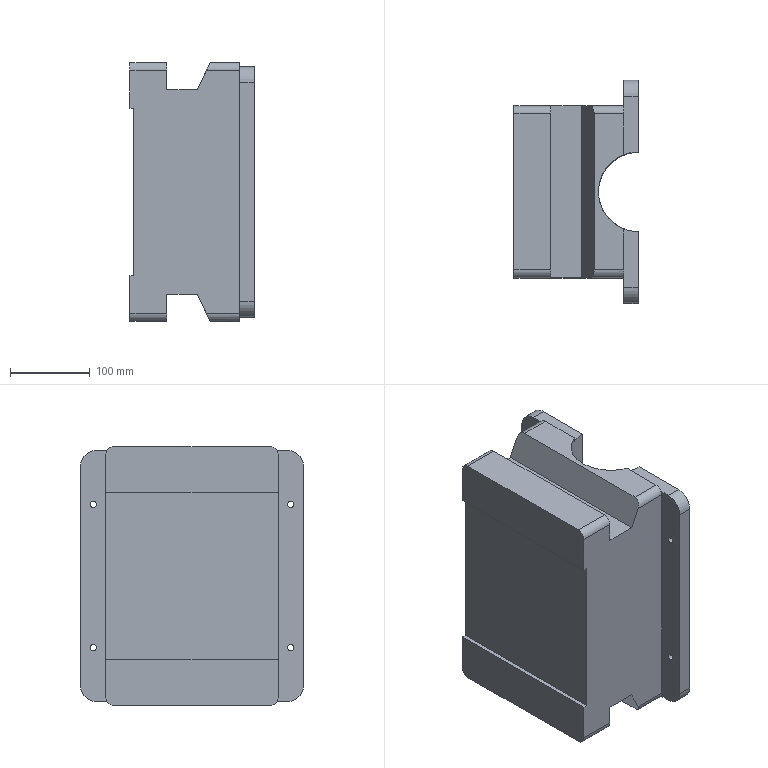Component | SolidWorks | Box-1 | 1 solid | 74 faces | box 156 x 280 x 325 mm | volume 4058266 mm3 | plane 40 | cylinder 34 | commonest cylinder face diameters 12 x8 8 x8 20 x8 40 x8 100 x2
build123d program:
from build123d import *

# Parameters (mm, degrees)
BOSS_EXTRUDE1_DEPTH = 18
BOSS_EXTRUDE2_DEPTH = 138
CUT_EXTRUDE1_DEPTH  = 141
CUT_EXTRUDE2_DEPTH  = 336.032
CUT_EXTRUDE3_DEPTH  = 336.032
CUT_EXTRUDE4_DEPTH  = 500
SKETCH7_R           = 4
SKETCH7_R_2         = 6
CUT_EXTRUDE5_DEPTH  = 20


with BuildPart() as part:
    # Sketch1 → Boss-Extrude1 (new body)
    with BuildSketch(Plane(origin=(0, 0, 0), x_dir=(0, 0, -1), z_dir=(1, 0, 0))):
        with BuildLine():
            Line((137.5, 140), (-137.5, 140))
            ThreePointArc((-137.5, 140), (-151.642, 134.142), (-157.5, 120))
            Line((-157.5, 120), (-157.5, -120))
            ThreePointArc((-157.5, -120), (-151.642, -134.142), (-137.5, -140))
            Line((-137.5, -140), (137.5, -140))
            ThreePointArc((137.5, -140), (151.642, -134.142), (157.5, -120))
            Line((157.5, -120), (157.5, 120))
            ThreePointArc((157.5, 120), (151.642, 134.142), (137.5, 140))
        make_face()
    extrude(amount=BOSS_EXTRUDE1_DEPTH)

    # Sketch2 → Boss-Extrude2 (add)
    with BuildSketch(Plane(origin=(18, 0, 0), x_dir=(0, 0, -1), z_dir=(1, 0, 0))):
        with BuildLine():
            Line((152.5, 108), (-152.5, 108))
            ThreePointArc((-152.5, 108), (-159.571, 105.071), (-162.5, 98))
            Line((-162.5, 98), (-162.5, -98))
            ThreePointArc((-162.5, -98), (-159.571, -105.071), (-152.5, -108))
            Line((-152.5, -108), (152.5, -108))
            ThreePointArc((152.5, -108), (159.571, -105.071), (162.5, -98))
            Line((162.5, -98), (162.5, 98))
            ThreePointArc((162.5, 98), (159.571, 105.071), (152.5, 108))
        make_face()
    extrude(amount=BOSS_EXTRUDE2_DEPTH)

    # Sketch3 → Cut-Extrude1 (cut)
    with BuildSketch(Plane.ZY):
        with BuildLine():
            Line((89.5, 96), (-89.5, 96))
            ThreePointArc((-89.5, 96), (-103.642, 90.142), (-109.5, 76))
            Line((-109.5, 76), (-109.5, -76))
            ThreePointArc((-109.5, -76), (-103.642, -90.142), (-89.5, -96))
            Line((-89.5, -96), (89.5, -96))
            ThreePointArc((89.5, -96), (103.642, -90.142), (109.5, -76))
            Line((109.5, -76), (109.5, 76))
            ThreePointArc((109.5, 76), (103.642, 90.142), (89.5, 96))
        make_face()
    extrude(amount=-CUT_EXTRUDE1_DEPTH, mode=Mode.SUBTRACT)

    # Sketch4 → Cut-Extrude2 (cut, through all)
    with BuildSketch(Plane.XZ.offset(108)):
        Polygon((156, 0), (156, 105), (151, 105), (151, -105), (156, -105), align=None)
    extrude(amount=-CUT_EXTRUDE2_DEPTH, mode=Mode.SUBTRACT)

    # Sketch5 → Cut-Extrude3 (cut, through all)
    with BuildSketch(Plane.XZ.offset(108)):
        Polygon((71.095, -128.5), (109.795, -128.5), (109.795, -162.5), (55.218, -162.5), align=None)
        Polygon((55.218, 162.5), (71.095, 128.5), (109.795, 128.5), (109.795, 162.5), align=None)
    extrude(amount=-CUT_EXTRUDE3_DEPTH, mode=Mode.SUBTRACT)

    # Sketch6 → Cut-Extrude4 (cut, symmetric)
    with BuildSketch(Plane(origin=(0, 0, -157.5), x_dir=(-1, 0, 0), z_dir=(0, 0, -1))):
        with BuildLine():
            Line((0, 50), (0, -50))
            ThreePointArc((0, -50), (-50, 0), (0, 50))
        make_face()
    extrude(amount=CUT_EXTRUDE4_DEPTH, both=True, mode=Mode.SUBTRACT)

    # Sketch7 → Cut-Extrude5 (cut)
    with BuildSketch(Plane.ZY):
        with Locations((-90, 124)):
            Circle(SKETCH7_R)
        with Locations((140, -65)):
            Circle(SKETCH7_R_2)
        with Locations(Location((90, 124, 0), (0, 0, 180))):
            Circle(SKETCH7_R)
        with Locations((90, -124)):
            Circle(SKETCH7_R)
        with Locations(Location((-90, -124, 0), (0, 0, 180))):
            Circle(SKETCH7_R)
        with Locations(Location((140, 65, 0), (0, 0, 180))):
            Circle(SKETCH7_R_2)
        with Locations((-140, 65)):
            Circle(SKETCH7_R_2)
        with Locations(Location((-140, -65, 0), (0, 0, 180))):
            Circle(SKETCH7_R_2)
    extrude(amount=-CUT_EXTRUDE5_DEPTH, mode=Mode.SUBTRACT)


solid = part.part

# Placed as in the assembly
solid = solid.moved(Location((35.733, 15.31, -110), (-180, 0, 180)))